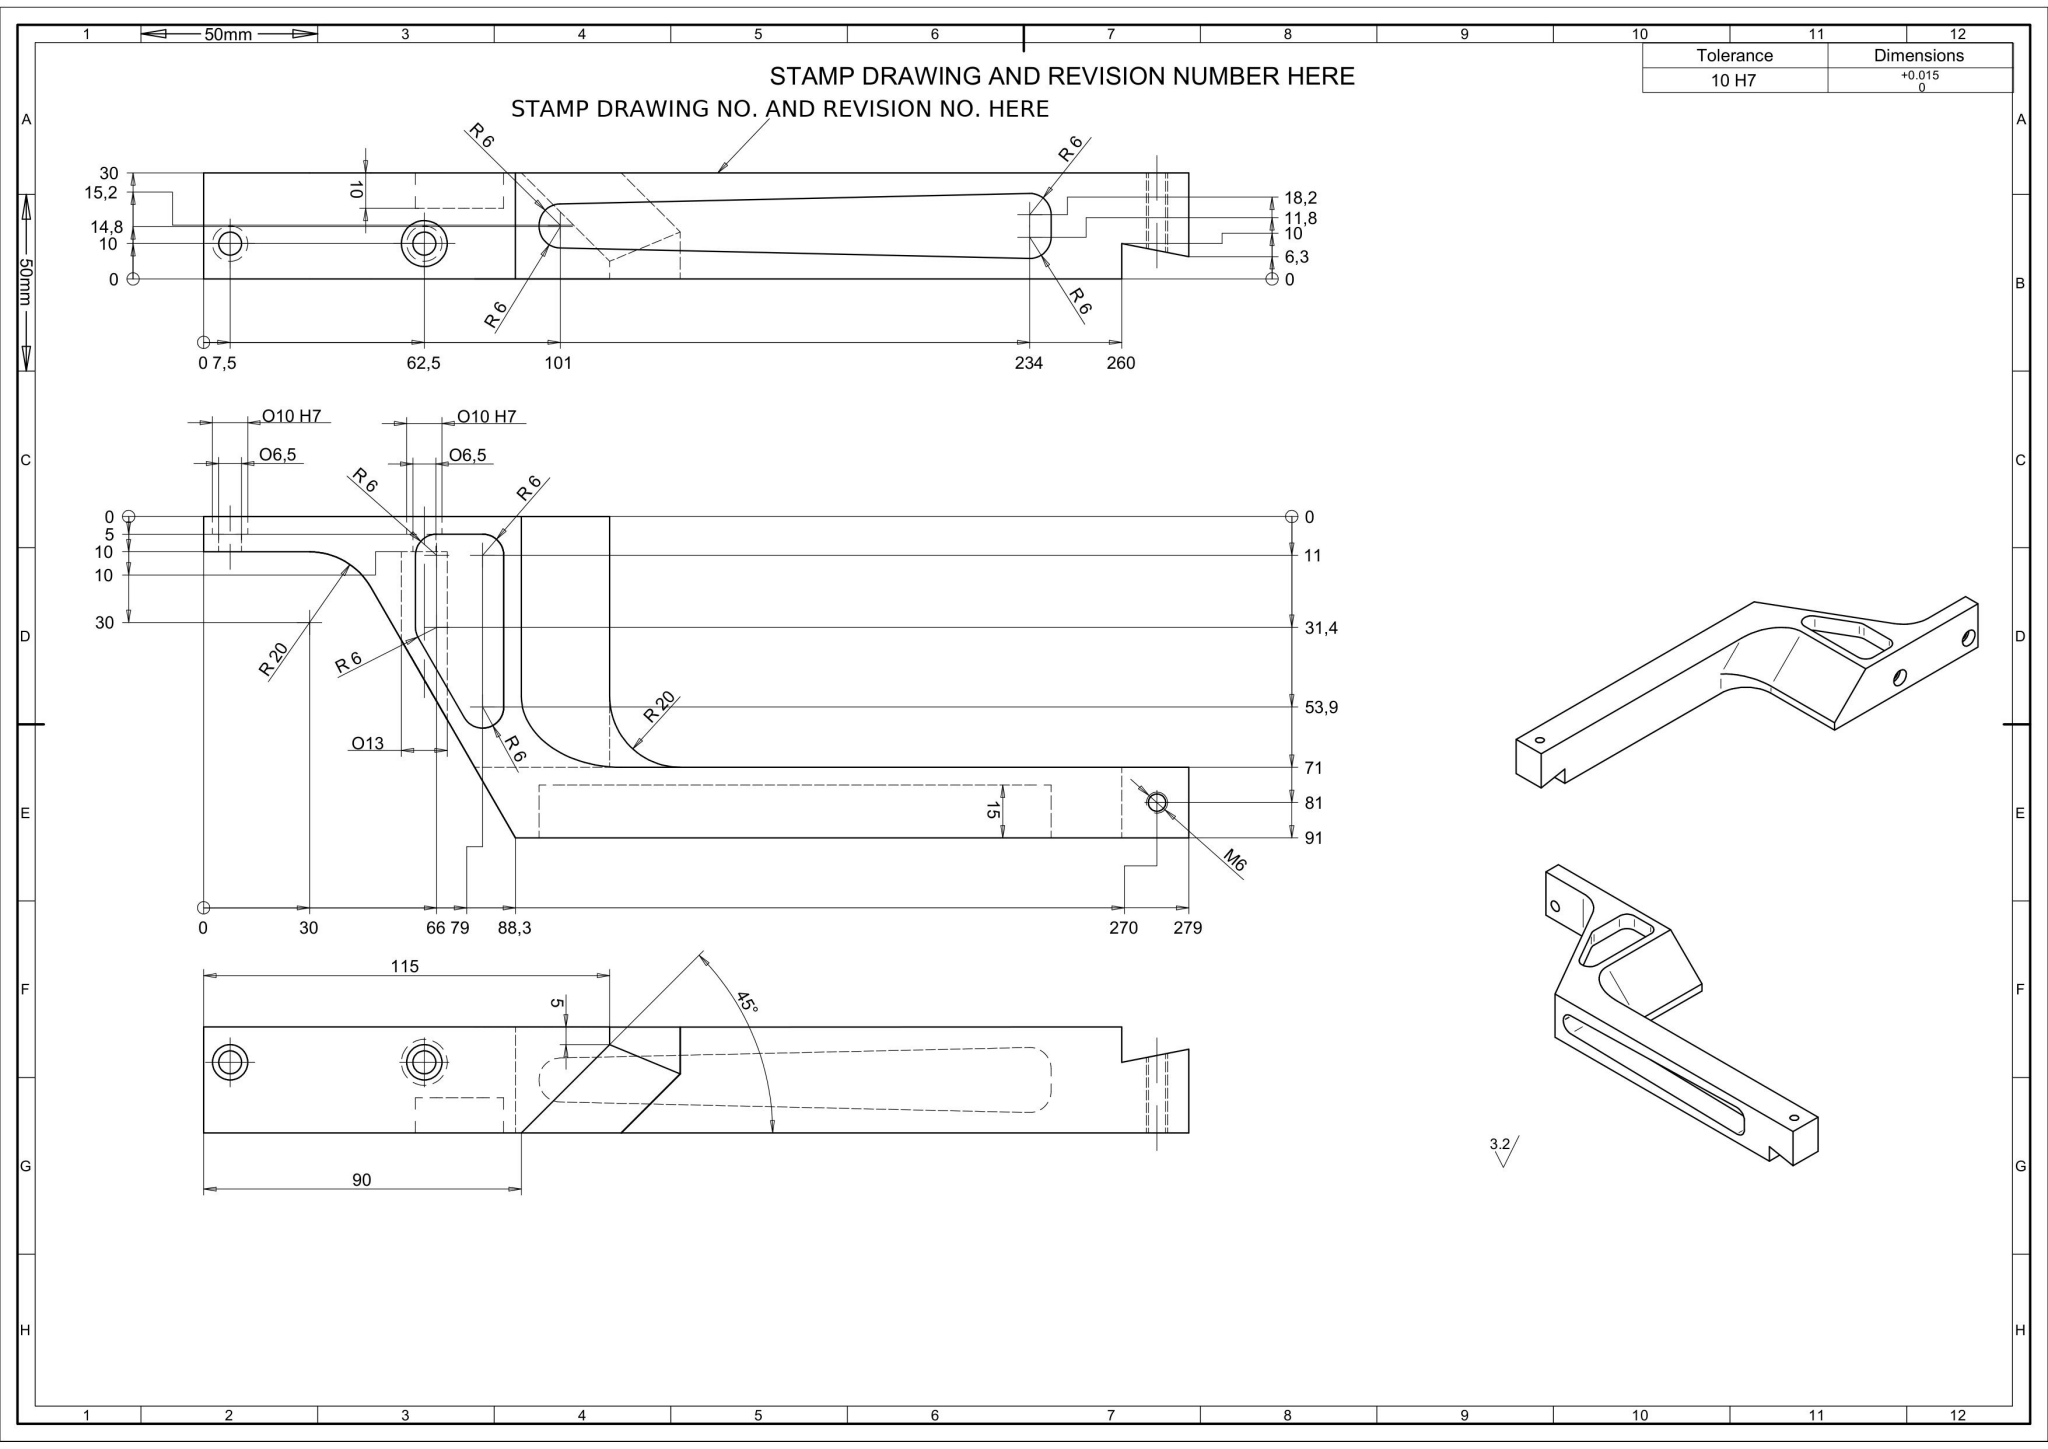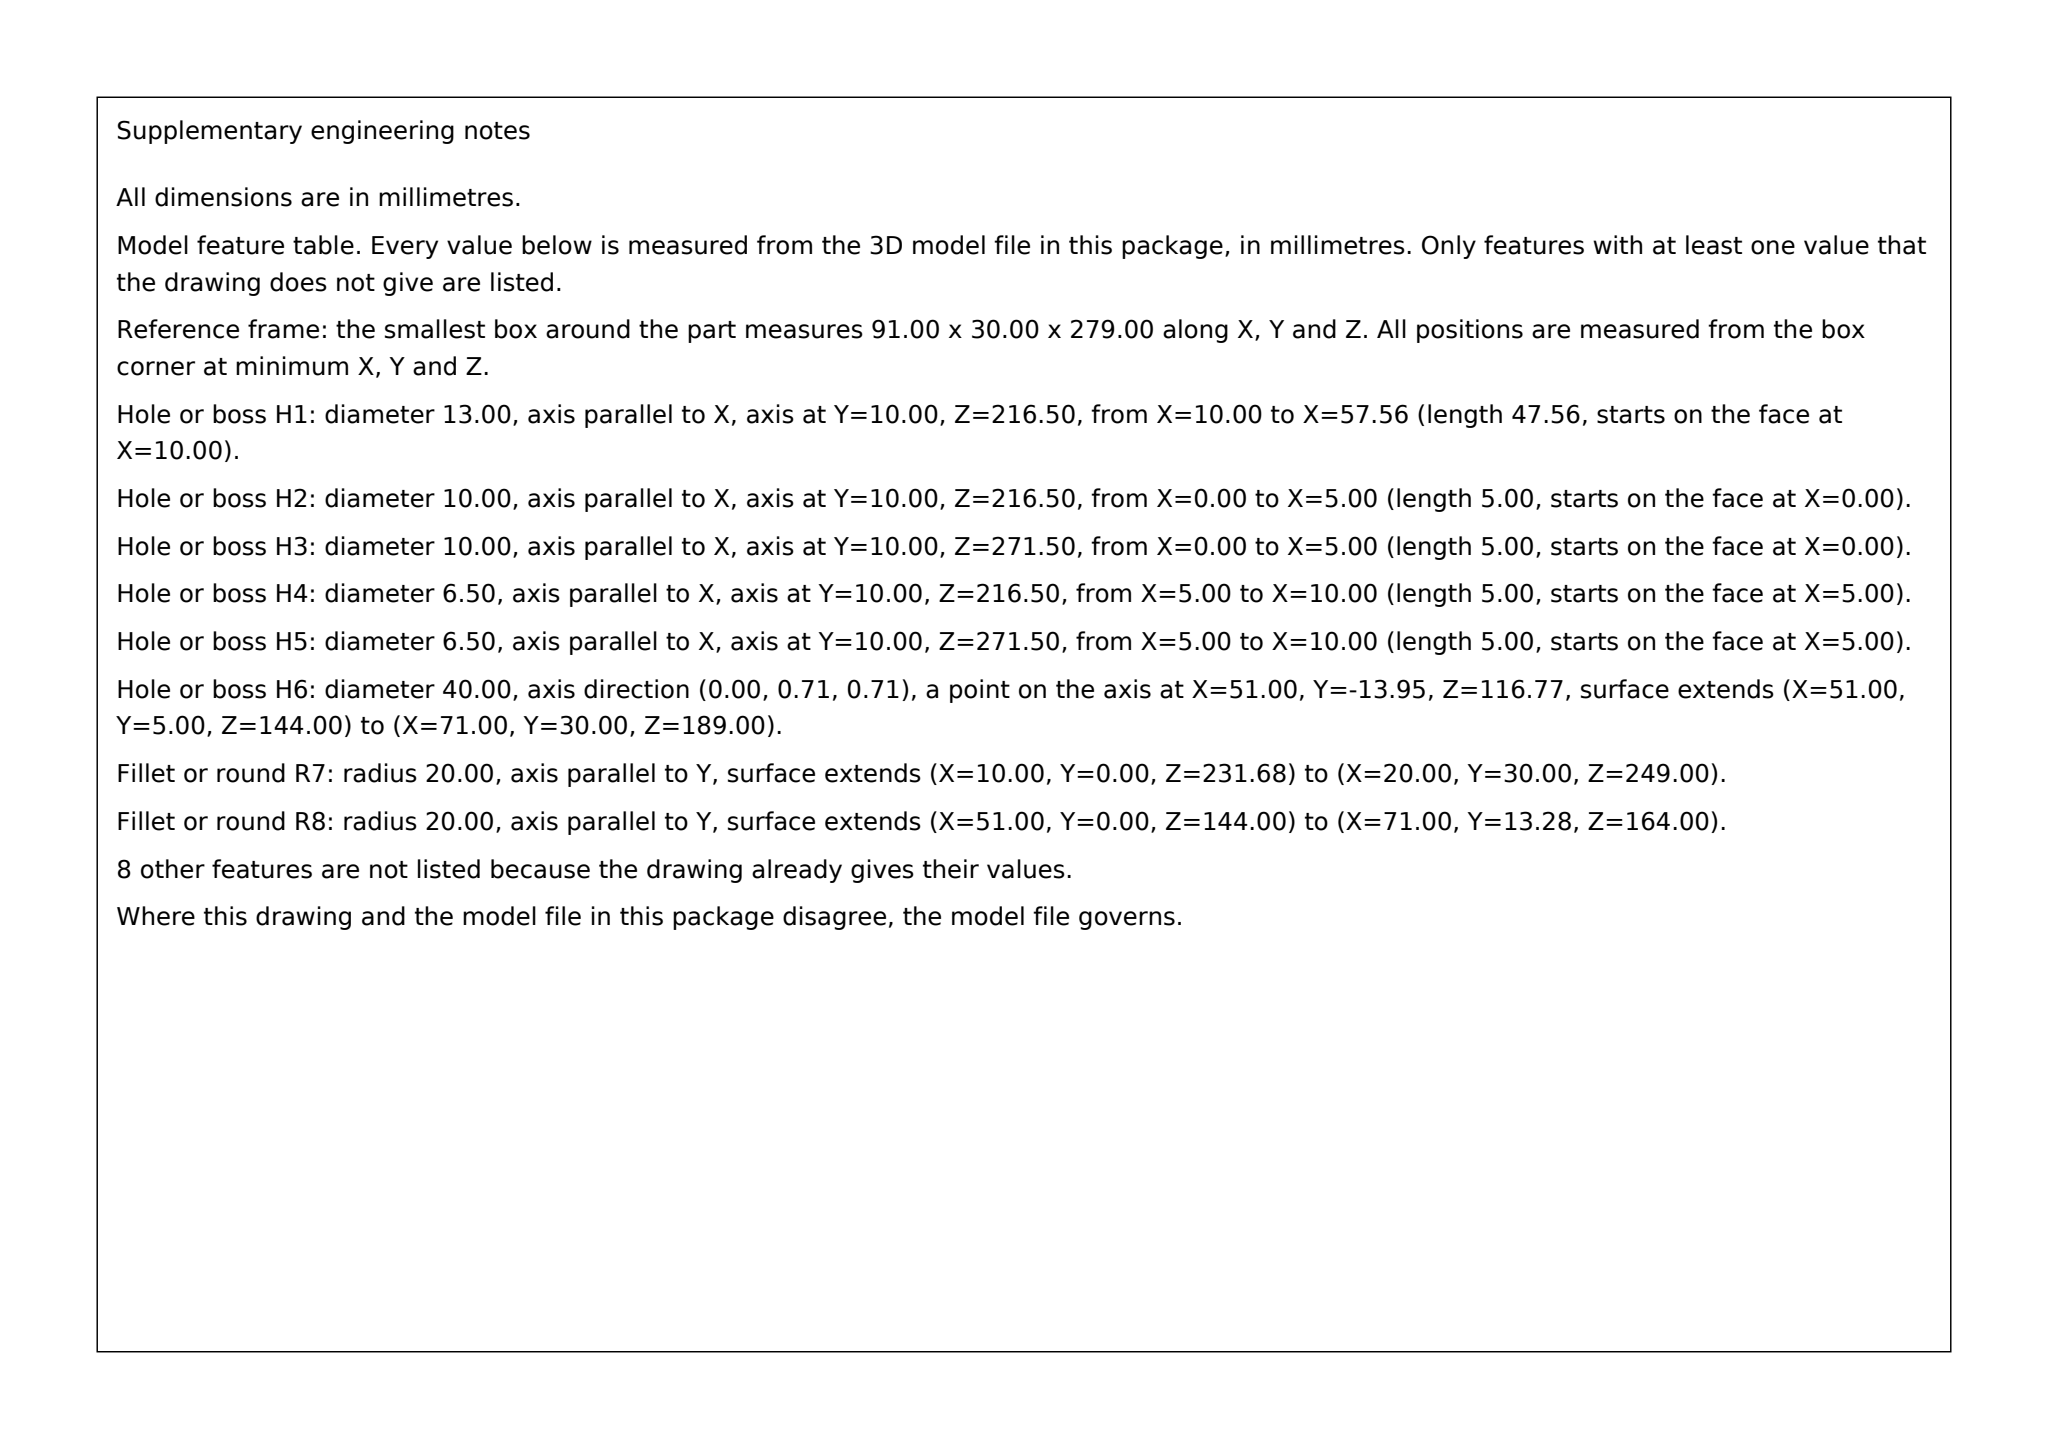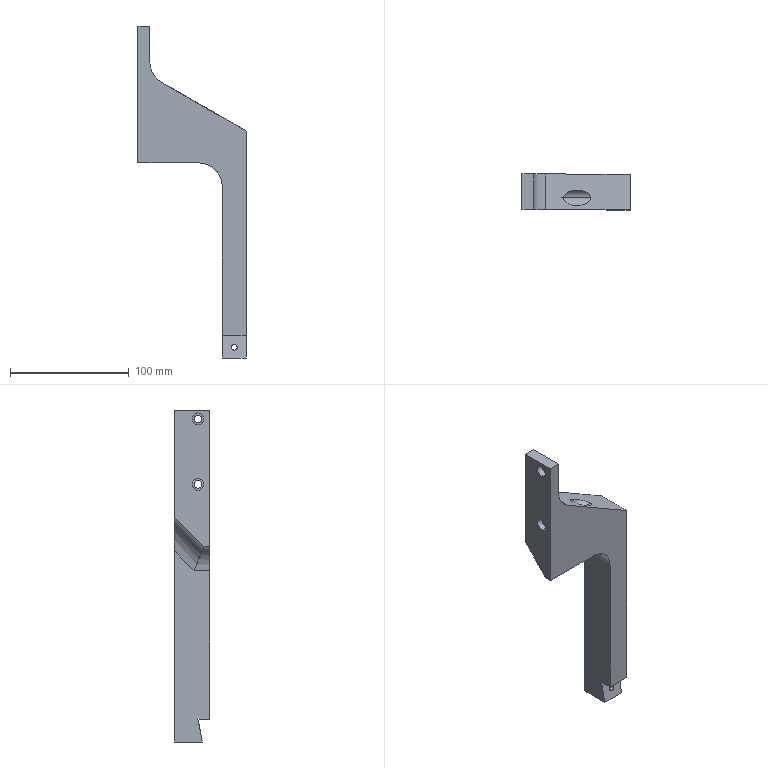Part | SolidWorks | mm | 1 solid | 48 faces | box 91 x 30 x 279 mm | volume 183010 mm3 | plane 25 | cylinder 23 | commonest cylinder face diameters 12 x8 6.5 x4 10 x4 40 x3 13 x2 4.917 x2